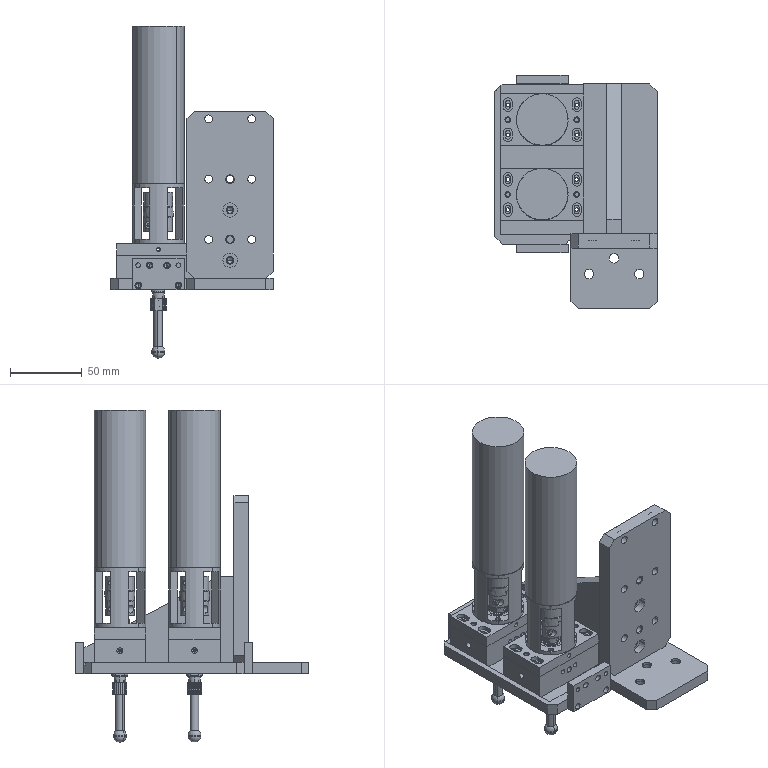Assembly | SolidWorks | mm | 35 component files | 35 solids | 1410 faces | box 113 x 162.5 x 231.3 mm | volume 559504 mm3 | cylinder 604 | plane 562 | cone 192 | spline 40 | torus 12 | commonest cylinder face diameters 3 x66 11 x42 8 x40 2.5 x36 3.3 x32 3.5 x32 5.5 x30 4.2 x26
Bill of materials:
03-MilledRib | 1 |  | Solid block with a tapered, roughly trapezoidal side profile: one tall flat end face, a top edge, a long sloped edge, and a short flat end at the narrow side.
03-MillingMaterialMotorMountingPlate | 1 |  | Flat rectangular plate with all four corners chamfered and a symmetric pattern of through holes.
03-SmallMotorFixingPlate | 1 | Plain Carbon Steel | Notched, roughly L-shaped flat plate with chamfered corners, two large rounded openings, and many smaller holes.
AdjustingPlate | 2 |  | Thick rectangular block with six round through holes of three sizes.
1.5KW-80-ER16A2 | 2 |  | Solid round cylinder with a short, stepped, smaller-diameter pin projecting from one end.
37bi-mpp70-3020 | 2 |  | Rectangular flange plate with a cylindrical boss projecting from one face, a large central bore, and slotted and round mounting holes.
37bi-mpp70-3021 | 2 |  | Short cylindrical sleeve with a through bore, two opposite flats, and longitudinal grooves on the outside.
37bi-mpp70-3022 | 2 |  | Long slender hollow tube with a collar near one end, a tapered end with an axial slit, and a small cross hole.
ConnectFastener2 | 2 |  | Cylindrical cage-style spacer: two annular end flanges, each with four holes, joined by a cylindrical wall with large rectangular windows.
FL678ZZ2 | 4 |  | Flanged bushing: a thin annular flange on top of a shorter-diameter cylindrical body, with a through bore.
M8Nut2 | 2 |  | Ring-shaped collar with a large through bore, two opposite flats, a radial hole in the side, and a short reduced-diameter step on one face.
M3-10_bo2 | 4 |  | Shape like a socket-head cap screw: a cylindrical head with a hexagonal socket and a plain cylindrical shank with a chamfered end.
MCOCG_spacer22 | 2 |  | Short, thick, ring-shaped (annular) disc with a central round through-bore. A straight rectangular slot is cut across the ring from one face, part of the way through the thickness. The outer diameter appears to have a slight step, so the slotted portion looks marginally larger than the rest.
MCOCG20-8_co2 | 4 |  | Cylindrical collar with a central round bore. A single radial slit runs from the bore out through the outer wall, so the ring is split. A small rectangular keyway-like notch is cut into the bore opposite the slit. A raised rectangular bar runs across the top face, and the slit cuts through the bar. A transverse hole with a counterbore or spot face passes into the side wall. The bottom outer edge appears to have a small chamfer.
SpacerBlock | 2 |  | Solid rectangular block with a large circular through-bore in the centre of the top face. The top face also has four elongated slots near the short ends (two at each end) and two small round holes, one between each pair of slots, that appear countersunk or counterbored. One long side face has three small holes, the middle one larger. One short end face has a single centred hole. The side holes appear blind, with conical drill-point bottoms.
Mates:
1. coincident | 03-SmallMotorFixingPlate-1 face at (30, 4, -162.197) dir (0, 0, 1) | 03-MillingMaterialMotorMountingPlate-1 face at (-30, 56, -162.197) dir (0, 0, -1)
2. coincident | 03-SmallMotorFixingPlate-1 face at (30, 4, -162.197) dir (1, 0, 0) | 03-MillingMaterialMotorMountingPlate-1 face at (30, 56, -162.197) dir (1, 0, 0)
3. coincident | 03-MillingMaterialMotorMountingPlate-1 face at (30, 56, -46.197) dir (0, 1, 0) | 03-MilledRib-1 face at (5, 56, -102.197) dir (0, -1, 0)
4. coincident | 03-SmallMotorFixingPlate-1 face at (30, 4, -162.197) dir (0, 0, 1) | 03-MilledRib-1 face at (5, 56, -162.197) dir (0, 0, -1)
5. concentric | 03-MillingMaterialMotorMountingPlate-1 face at (0, 46, -149.697) dir (0, -1, 0) r 2.75 | 03-MilledRib-1 face at (0, 56, -149.697) dir (0, -1, 0) r 2.1
6. coincident | 03-MillingCutterHead-1 face at (-37.252, 100.647, -179.997) dir (0, 0, 1) | 03-MillingCutterHead-2 face at (-29.266, 140.661, -179.997) dir (0, 0, 1)
7. coincident | 03-SmallMotorFixingPlate-1 face at (-80, 160.5, -162.197) dir (0, 1, 0) | 03-MilledRib-1 face at (5, 160.5, -162.197) dir (0, 1, 0)
8. coincident | 03-SmallMotorFixingPlate-1 face at (-80, 160.5, -164.197) dir (0, 0, 1) | SpacerBlock-1 face at (-21, 117.5, -164.197) dir (0, 0, -1)
9. coincident | SpacerBlock-1 face at (-21, 117.5, -146.197) dir (0, 0, 1) | MotorAssemblyWhen2-1/37bi-mpp70-3020-1 face at (-50, 135.5, -146.197) dir (0, 0, -1)
10. coincident | SpacerBlock-1 face at (-79, 153.5, -146.197) dir (0, 1, 0) | MotorAssemblyWhen2-1/37bi-mpp70-3020-1 face at (-79, 153.5, -146.197) dir (0, 1, 0)
11. coincident | SpacerBlock-1 face at (-79, 153.5, -146.197) dir (-1, 0, 0) | MotorAssemblyWhen2-1/37bi-mpp70-3020-1 face at (-79, 117.5, -146.197) dir (-1, 0, 0)
12. coincident | SpacerBlock-2 face at (-79, 101.5, -146.197) dir (0, 1, 0) | MotorAssemblyWhen2-2/37bi-mpp70-3020-1 face at (-79, 101.5, -146.197) dir (0, 1, 0)
13. coincident | SpacerBlock-2 face at (-79, 101.5, -146.197) dir (-1, 0, 0) | MotorAssemblyWhen2-2/37bi-mpp70-3020-1 face at (-79, 65.5, -146.197) dir (-1, 0, 0)
14. coincident | 03-SmallMotorFixingPlate-1 face at (-21, 160.5, -164.197) dir (-1, 0, 0) | SpacerBlock-2 face at (-21, 101.5, -146.197) dir (1, 0, 0)
15. coincident | SpacerBlock-2 face at (-21, 65.5, -146.197) dir (0, 0, 1) | MotorAssemblyWhen2-2/37bi-mpp70-3020-1 face at (-50, 83.5, -146.197) dir (0, 0, -1)
16. coincident | 03-SmallMotorFixingPlate-1 face at (-80, 160.5, -164.197) dir (0, 0, 1) | SpacerBlock-2 face at (-21, 65.5, -164.197) dir (0, 0, -1)
17. coincident | 03-SmallMotorFixingPlate-1 face at (-21, 160.5, -164.197) dir (-1, 0, 0) | SpacerBlock-1 face at (-21, 153.5, -146.197) dir (1, 0, 0)
18. concentric | 03-MillingCutterHead-2 face at (-50, 135.5, -209.997) dir (0, 0, 1) r 3 | MotorAssemblyWhen2-1/37bi-mpp70-3021-1 face at (-50, 135.5, -175.097) dir (0, 0, -1) r 3.15
19. concentric | 03-MillingCutterHead-1 face at (-50, 83.5, -209.997) dir (0, 0, 1) r 3 | MotorAssemblyWhen2-2/37bi-mpp70-3021-1 face at (-50, 83.5, -175.097) dir (0, 0, -1) r 3.15
20. distance | MotorAssemblyWhen2-1/37bi-mpp70-3021-1 face at (-50, 135.5, -184.997) dir (0, 0, -1) | 03-MillingCutterHead-2 face at (-29.266, 140.661, -179.997) dir (0, 0, 1)
21. coincident | 03-SmallMotorFixingPlate-1 face at (-80, 160.5, -162.197) dir (0, 1, 0) | AdjustingPlate-1 face at (-68, 160.5, -148.197) dir (0, -1, 0)
22. concentric | 03-SmallMotorFixingPlate-1 face at (-64, 160.5, -167.197) dir (0, 1, 0) r 1.65 | AdjustingPlate-1 face at (-64, 160.5, -167.197) dir (0, -1, 0) r 2.25
23. coincident | 03-SmallMotorFixingPlate-1 face at (-80, 49, -170.197) dir (0, -1, 0) | AdjustingPlate-2 face at (-68, 49, -148.197) dir (0, 1, 0)
24. concentric | 03-SmallMotorFixingPlate-1 face at (-64, 49, -167.197) dir (0, -1, 0) r 1.65 | AdjustingPlate-2 face at (-64, 43, -167.197) dir (0, -1, 0) r 2.25
25. distance | MotorAssemblyWhen2-1/37bi-mpp70-3020-1 face at (-79, 153.5, -146.197) dir (0, 1, 0) | 03-SmallMotorFixingPlate-1 face at (-80, 160.5, -162.197) dir (0, 1, 0)
26. distance | MotorAssemblyWhen2-2/37bi-mpp70-3020-1 face at (-79, 101.5, -146.197) dir (0, 1, 0) | MotorAssemblyWhen2-1/37bi-mpp70-3020-1 face at (-21, 117.5, -146.197) dir (0, -1, 0)